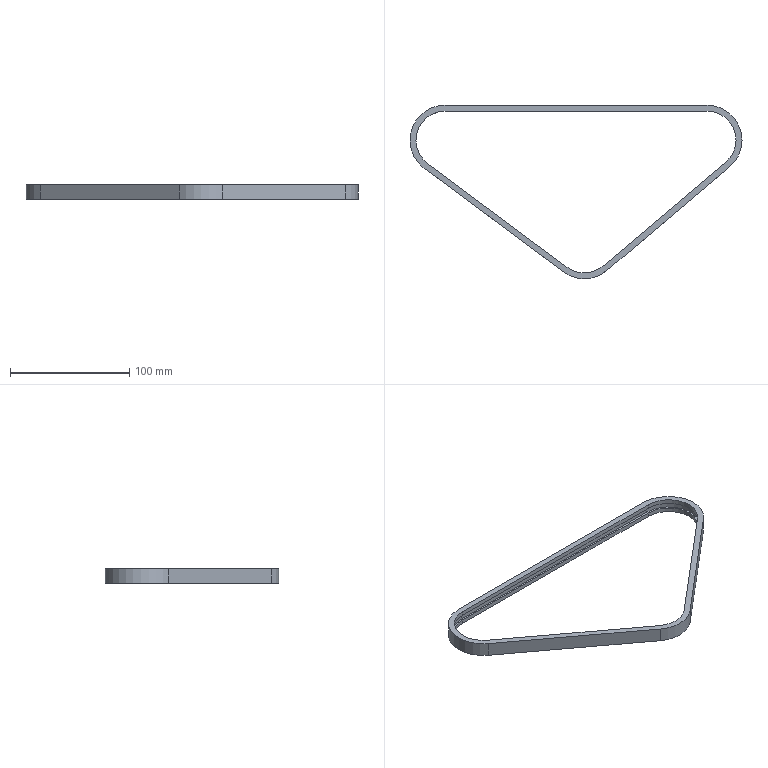Component | SolidWorks | LD101-02--Q1000-Q16-1.SLDQ1SM-1_LD101-02-Chain35B-1 | 1 solid | 32 faces | box 278.82 x 145.82 x 12 mm | volume 35184 mm3 | cylinder 16 | plane 16 | commonest cylinder face diameters 48.82 x8 52 x4 58.82 x4 | material 45
build123d program:
from build123d import *

# Parameters (mm, degrees)
EXTRUDE_THIN1_DEPTH            = 6
CHAIN_PLATE_GAP_SPROCKET_DEPTH = 2.385


with BuildPart() as part:
    # Sketch1_2 → Extrude-Thin1 (new, symmetric)
    with BuildSketch(Plane.XY):
        with BuildLine():
            Line((10.549, -110.6), (127.549, -23.6))
            ThreePointArc((127.549, -23.6), (137.92, 9.243), (110, 29.41))
            Line((110, 29.41), (-110, 29.41))
            ThreePointArc((-110, 29.41), (-137.62, 10.104), (-128.978, -22.468))
            Line((-128.978, -22.468), (-25.978, -109.468))
            ThreePointArc((-25.978, -109.468), (-7.912, -116.396), (10.549, -110.6))
        make_face()
        with BuildLine():
            Line((7.566, -106.588), (124.566, -19.588))
            ThreePointArc((124.566, -19.588), (133.173, 7.671), (110, 24.41))
            Line((110, 24.41), (-110, 24.41))
            ThreePointArc((-110, 24.41), (-132.924, 8.386), (-125.751, -18.648))
            Line((-125.751, -18.648), (-22.751, -105.648))
            ThreePointArc((-22.751, -105.648), (-7.757, -111.398), (7.566, -106.588))
        make_face(mode=Mode.SUBTRACT)
    extrude(amount=EXTRUDE_THIN1_DEPTH, both=True)

    # Sketch1_2 2 → Chain Plate Gap-Sprocket (cut, symmetric)
    with BuildSketch(Plane.XY):
        with BuildLine():
            Line((8.514, -107.864), (125.514, -20.864))
            ThreePointArc((125.514, -20.864), (134.683, 8.171), (110, 26))
            Line((110, 26), (-110, 26))
            ThreePointArc((-110, 26), (-134.418, 8.932), (-126.777, -19.863))
            Line((-126.777, -19.863), (-23.777, -106.863))
            ThreePointArc((-23.777, -106.863), (-7.806, -112.988), (8.514, -107.864))
        make_face()
        with BuildLine():
            Line((6.617, -105.312), (123.617, -18.312))
            ThreePointArc((123.617, -18.312), (131.664, 7.172), (110, 22.82))
            Line((110, 22.82), (-110, 22.82))
            ThreePointArc((-110, 22.82), (-131.431, 7.84), (-124.725, -17.433))
            Line((-124.725, -17.433), (-21.725, -104.433))
            ThreePointArc((-21.725, -104.433), (-7.707, -109.809), (6.617, -105.312))
        make_face(mode=Mode.SUBTRACT)
    extrude(amount=CHAIN_PLATE_GAP_SPROCKET_DEPTH, both=True, mode=Mode.SUBTRACT)


solid = part.part

# Placed as in the assembly
solid = solid.moved(Location((-760.29, 11.103, -50.893), (-180, 0, 180)))
STEP:
#1=COLOUR_RGB('',0.7922,0.8196,0.9333);
#2=FILL_AREA_STYLE_COLOUR('',#1);
#3=FILL_AREA_STYLE('',(#2));
#4=SURFACE_STYLE_FILL_AREA(#3);
#5=SURFACE_SIDE_STYLE('',(#4));
#6=SURFACE_STYLE_USAGE(.BOTH.,#5);
#7=PRESENTATION_STYLE_ASSIGNMENT((#6));
#8=CARTESIAN_POINT('',(-35.287,0.4371,-1.91));
#9=VERTEX_POINT('',#8);
#10=CARTESIAN_POINT('',(-34.263,1.461,-1.91));
#11=VERTEX_POINT('',#10);
#12=CARTESIAN_POINT('',(-34.263,0.4371,-1.91));
#13=DIRECTION('',(0.,0.,-1.));
#14=DIRECTION('',(-1.,-0.,-0.));
#15=AXIS2_PLACEMENT_3D('',#12,#13,#14);
#16=CIRCLE('',#15,1.024);
#17=EDGE_CURVE('',#9,#11,#16,.T.);
#18=ORIENTED_EDGE('',*,*,#17,.F.);
#19=CARTESIAN_POINT('',(-35.287,0.4371,-2.098));
#20=VERTEX_POINT('',#19);
#21=CARTESIAN_POINT('',(-35.287,0.4371,-1.91));
#22=DIRECTION('',(0.,0.,-1.));
#23=VECTOR('',#22,39.37);
#24=LINE('',#21,#23);
#25=EDGE_CURVE('',#9,#20,#24,.T.);
#26=ORIENTED_EDGE('',*,*,#25,.T.);
#27=CARTESIAN_POINT('',(-34.263,1.461,-2.098));
#28=VERTEX_POINT('',#27);
#29=CARTESIAN_POINT('',(-34.263,0.4371,-2.098));
#30=DIRECTION('',(0.,0.,-1.));
#31=DIRECTION('',(-1.,-0.,-0.));
#32=AXIS2_PLACEMENT_3D('',#29,#30,#31);
#33=CIRCLE('',#32,1.024);
#34=EDGE_CURVE('',#20,#28,#33,.T.);
#35=ORIENTED_EDGE('',*,*,#34,.T.);
#36=CARTESIAN_POINT('',(-34.263,1.461,-1.91));
#37=DIRECTION('',(0.,0.,-1.));
#38=VECTOR('',#37,39.37);
#39=LINE('',#36,#38);
#40=EDGE_CURVE('',#11,#28,#39,.T.);
#41=ORIENTED_EDGE('',*,*,#40,.F.);
#42=EDGE_LOOP('',(#18,#26,#35,#41));
#43=FACE_OUTER_BOUND('',#42,.T.);
#44=CARTESIAN_POINT('',(-34.263,0.4371,-1.91));
#45=DIRECTION('',(0.,0.,-1.));
#46=DIRECTION('',(-1.,-0.,-0.));
#47=AXIS2_PLACEMENT_3D('',#44,#45,#46);
#48=CYLINDRICAL_SURFACE('',#47,1.024);
#49=ADVANCED_FACE('',(#43),#48,.F.);
#50=CARTESIAN_POINT('',(-25.602,1.398,-2.24));
#51=VERTEX_POINT('',#50);
#52=CARTESIAN_POINT('',(-24.641,0.4371,-2.24));
#53=VERTEX_POINT('',#52);
#54=CARTESIAN_POINT('',(-25.602,0.4371,-2.24));
#55=DIRECTION('',(0.,0.,-1.));
#56=DIRECTION('',(-1.,-0.,-0.));
#57=AXIS2_PLACEMENT_3D('',#54,#55,#56);
#58=CIRCLE('',#57,0.961);
#59=EDGE_CURVE('',#51,#53,#58,.T.);
#60=ORIENTED_EDGE('',*,*,#59,.T.);
#61=CARTESIAN_POINT('',(-24.641,0.4371,-2.098));
#62=VERTEX_POINT('',#61);
#63=CARTESIAN_POINT('',(-24.641,0.4371,-2.24));
#64=DIRECTION('',(-0.,-0.,1.));
#65=VECTOR('',#64,39.37);
#66=LINE('',#63,#65);
#67=EDGE_CURVE('',#53,#62,#66,.T.);
#68=ORIENTED_EDGE('',*,*,#67,.T.);
#69=CARTESIAN_POINT('',(-25.602,1.398,-2.098));
#70=VERTEX_POINT('',#69);
#71=CARTESIAN_POINT('',(-25.602,0.4371,-2.098));
#72=DIRECTION('',(0.,0.,-1.));
#73=DIRECTION('',(-1.,-0.,-0.));
#74=AXIS2_PLACEMENT_3D('',#71,#72,#73);
#75=CIRCLE('',#74,0.961);
#76=EDGE_CURVE('',#70,#62,#75,.T.);
#77=ORIENTED_EDGE('',*,*,#76,.F.);
#78=CARTESIAN_POINT('',(-25.602,1.398,-2.24));
#79=DIRECTION('',(-0.,-0.,1.));
#80=VECTOR('',#79,39.37);
#81=LINE('',#78,#80);
#82=EDGE_CURVE('',#51,#70,#81,.T.);
#83=ORIENTED_EDGE('',*,*,#82,.F.);
#84=EDGE_LOOP('',(#60,#68,#77,#83));
#85=FACE_OUTER_BOUND('',#84,.T.);
#86=CARTESIAN_POINT('',(-25.602,0.4371,-2.24));
#87=DIRECTION('',(-0.,-0.,1.));
#88=DIRECTION('',(1.,0.,0.));
#89=AXIS2_PLACEMENT_3D('',#86,#87,#88);
#90=CYLINDRICAL_SURFACE('',#89,0.961);
#91=ADVANCED_FACE('',(#85),#90,.F.);
#92=CARTESIAN_POINT('',(-24.444,0.4371,-2.24));
#93=VERTEX_POINT('',#92);
#94=CARTESIAN_POINT('',(-24.855,-0.4474,-2.24));
#95=VERTEX_POINT('',#94);
#96=CARTESIAN_POINT('',(-25.602,0.4371,-2.24));
#97=DIRECTION('',(0.,0.,-1.));
#98=DIRECTION('',(-1.,-0.,-0.));
#99=AXIS2_PLACEMENT_3D('',#96,#97,#98);
#100=CIRCLE('',#99,1.158);
#101=EDGE_CURVE('',#93,#95,#100,.T.);
#102=ORIENTED_EDGE('',*,*,#101,.F.);
#103=CARTESIAN_POINT('',(-24.444,0.4371,-1.767));
#104=VERTEX_POINT('',#103);
#105=CARTESIAN_POINT('',(-24.444,0.4371,-2.24));
#106=DIRECTION('',(-0.,-0.,1.));
#107=VECTOR('',#106,39.37);
#108=LINE('',#105,#107);
#109=EDGE_CURVE('',#93,#104,#108,.T.);
#110=ORIENTED_EDGE('',*,*,#109,.T.);
#111=CARTESIAN_POINT('',(-24.855,-0.4474,-1.767));
#112=VERTEX_POINT('',#111);
#113=CARTESIAN_POINT('',(-25.602,0.4371,-1.767));
#114=DIRECTION('',(0.,0.,-1.));
#115=DIRECTION('',(-1.,-0.,-0.));
#116=AXIS2_PLACEMENT_3D('',#113,#114,#115);
#117=CIRCLE('',#116,1.158);
#118=EDGE_CURVE('',#104,#112,#117,.T.);
#119=ORIENTED_EDGE('',*,*,#118,.T.);
#120=CARTESIAN_POINT('',(-24.855,-0.4474,-2.24));
#121=DIRECTION('',(-0.,-0.,1.));
#122=VECTOR('',#121,39.37);
#123=LINE('',#120,#122);
#124=EDGE_CURVE('',#95,#112,#123,.T.);
#125=ORIENTED_EDGE('',*,*,#124,.F.);
#126=EDGE_LOOP('',(#102,#110,#119,#125));
#127=FACE_OUTER_BOUND('',#126,.T.);
#128=CARTESIAN_POINT('',(-25.602,0.4371,-2.24));
#129=DIRECTION('',(-0.,-0.,1.));
#130=DIRECTION('',(1.,0.,0.));
#131=AXIS2_PLACEMENT_3D('',#128,#129,#130);
#132=CYLINDRICAL_SURFACE('',#131,1.158);
#133=ADVANCED_FACE('',(#127),#132,.T.);
#134=CARTESIAN_POINT('',(-25.602,1.398,-1.91));
#135=VERTEX_POINT('',#134);
#136=CARTESIAN_POINT('',(-24.641,0.4371,-1.91));
#137=VERTEX_POINT('',#136);
#138=CARTESIAN_POINT('',(-25.602,0.4371,-1.91));
#139=DIRECTION('',(0.,0.,-1.));
#140=DIRECTION('',(-1.,-0.,-0.));
#141=AXIS2_PLACEMENT_3D('',#138,#139,#140);
#142=CIRCLE('',#141,0.961);
#143=EDGE_CURVE('',#135,#137,#142,.T.);
#144=ORIENTED_EDGE('',*,*,#143,.T.);
#145=CARTESIAN_POINT('',(-24.641,0.4371,-1.767));
#146=VERTEX_POINT('',#145);
#147=CARTESIAN_POINT('',(-24.641,0.4371,-2.24));
#148=DIRECTION('',(-0.,-0.,1.));
#149=VECTOR('',#148,39.37);
#150=LINE('',#147,#149);
#151=EDGE_CURVE('',#137,#146,#150,.T.);
#152=ORIENTED_EDGE('',*,*,#151,.T.);
#153=CARTESIAN_POINT('',(-25.602,1.398,-1.767));
#154=VERTEX_POINT('',#153);
#155=CARTESIAN_POINT('',(-25.602,0.4371,-1.767));
#156=DIRECTION('',(0.,0.,-1.));
#157=DIRECTION('',(-1.,-0.,-0.));
#158=AXIS2_PLACEMENT_3D('',#155,#156,#157);
#159=CIRCLE('',#158,0.961);
#160=EDGE_CURVE('',#154,#146,#159,.T.);
#161=ORIENTED_EDGE('',*,*,#160,.F.);
#162=CARTESIAN_POINT('',(-25.602,1.398,-2.24));
#163=DIRECTION('',(-0.,-0.,1.));
#164=VECTOR('',#163,39.37);
#165=LINE('',#162,#164);
#166=EDGE_CURVE('',#135,#154,#165,.T.);
#167=ORIENTED_EDGE('',*,*,#166,.F.);
#168=EDGE_LOOP('',(#144,#152,#161,#167));
#169=FACE_OUTER_BOUND('',#168,.T.);
#170=CARTESIAN_POINT('',(-25.602,0.4371,-2.24));
#171=DIRECTION('',(-0.,-0.,1.));
#172=DIRECTION('',(1.,0.,0.));
#173=AXIS2_PLACEMENT_3D('',#170,#171,#172);
#174=CYLINDRICAL_SURFACE('',#173,0.961);
#175=ADVANCED_FACE('',(#169),#174,.F.);
#176=CARTESIAN_POINT('',(-29.037,-3.722,-1.91));
#177=VERTEX_POINT('',#176);
#178=CARTESIAN_POINT('',(-29.037,-3.722,-1.767));
#179=VERTEX_POINT('',#178);
#180=CARTESIAN_POINT('',(-29.037,-3.722,-2.24));
#181=DIRECTION('',(-0.,-0.,1.));
#182=VECTOR('',#181,39.37);
#183=LINE('',#180,#182);
#184=EDGE_CURVE('',#177,#179,#183,.T.);
#185=ORIENTED_EDGE('',*,*,#184,.F.);
#186=CARTESIAN_POINT('',(-30.231,-3.759,-1.91));
#187=VERTEX_POINT('',#186);
#188=CARTESIAN_POINT('',(-29.657,-2.988,-1.91));
#189=DIRECTION('',(0.,0.,-1.));
#190=DIRECTION('',(-1.,0.,-0.));
#191=AXIS2_PLACEMENT_3D('',#188,#189,#190);
#192=CIRCLE('',#191,0.961);
#193=EDGE_CURVE('',#177,#187,#192,.T.);
#194=ORIENTED_EDGE('',*,*,#193,.T.);
#195=CARTESIAN_POINT('',(-30.231,-3.759,-1.767));
#196=VERTEX_POINT('',#195);
#197=CARTESIAN_POINT('',(-30.231,-3.759,-2.24));
#198=DIRECTION('',(-0.,-0.,1.));
#199=VECTOR('',#198,39.37);
#200=LINE('',#197,#199);
#201=EDGE_CURVE('',#187,#196,#200,.T.);
#202=ORIENTED_EDGE('',*,*,#201,.T.);
#203=CARTESIAN_POINT('',(-29.657,-2.988,-1.767));
#204=DIRECTION('',(0.,0.,-1.));
#205=DIRECTION('',(-1.,0.,-0.));
#206=AXIS2_PLACEMENT_3D('',#203,#204,#205);
#207=CIRCLE('',#206,0.961);
#208=EDGE_CURVE('',#179,#196,#207,.T.);
#209=ORIENTED_EDGE('',*,*,#208,.F.);
#210=EDGE_LOOP('',(#185,#194,#202,#209));
#211=FACE_OUTER_BOUND('',#210,.T.);
#212=CARTESIAN_POINT('',(-29.657,-2.988,-2.24));
#213=DIRECTION('',(-0.,-0.,1.));
#214=DIRECTION('',(1.,0.,0.));
#215=AXIS2_PLACEMENT_3D('',#212,#213,#214);
#216=CYLINDRICAL_SURFACE('',#215,0.961);
#217=ADVANCED_FACE('',(#211),#216,.F.);
#218=ORIENTED_EDGE('',*,*,#201,.F.);
#219=CARTESIAN_POINT('',(-34.837,-0.3341,-1.91));
#220=VERTEX_POINT('',#219);
#221=CARTESIAN_POINT('',(-30.231,-3.759,-1.91));
#222=DIRECTION('',(-0.8025,0.5967,-0.));
#223=VECTOR('',#222,39.37);
#224=LINE('',#221,#223);
#225=EDGE_CURVE('',#187,#220,#224,.T.);
#226=ORIENTED_EDGE('',*,*,#225,.T.);
#227=CARTESIAN_POINT('',(-34.837,-0.3341,-1.767));
#228=VERTEX_POINT('',#227);
#229=CARTESIAN_POINT('',(-34.837,-0.3341,-2.24));
#230=DIRECTION('',(-0.,-0.,1.));
#231=VECTOR('',#230,39.37);
#232=LINE('',#229,#231);
#233=EDGE_CURVE('',#220,#228,#232,.T.);
#234=ORIENTED_EDGE('',*,*,#233,.T.);
#235=CARTESIAN_POINT('',(-30.231,-3.759,-1.767));
#236=DIRECTION('',(-0.8025,0.5967,-0.));
#237=VECTOR('',#236,39.37);
#238=LINE('',#235,#237);
#239=EDGE_CURVE('',#196,#228,#238,.T.);
#240=ORIENTED_EDGE('',*,*,#239,.F.);
#241=EDGE_LOOP('',(#218,#226,#234,#240));
#242=FACE_OUTER_BOUND('',#241,.T.);
#243=CARTESIAN_POINT('',(-30.231,-3.759,-2.24));
#244=DIRECTION('',(0.5967,0.8025,0.));
#245=DIRECTION('',(0.8025,-0.5967,0.));
#246=AXIS2_PLACEMENT_3D('',#243,#244,#245);
#247=PLANE('',#246);
#248=ADVANCED_FACE('',(#242),#247,.T.);
#249=ORIENTED_EDGE('',*,*,#233,.F.);
#250=CARTESIAN_POINT('',(-34.263,1.398,-1.91));
#251=VERTEX_POINT('',#250);
#252=CARTESIAN_POINT('',(-34.263,0.4371,-1.91));
#253=DIRECTION('',(0.,0.,-1.));
#254=DIRECTION('',(-1.,-0.,-0.));
#255=AXIS2_PLACEMENT_3D('',#252,#253,#254);
#256=CIRCLE('',#255,0.961);
#257=EDGE_CURVE('',#220,#251,#256,.T.);
#258=ORIENTED_EDGE('',*,*,#257,.T.);
#259=CARTESIAN_POINT('',(-34.263,1.398,-1.767));
#260=VERTEX_POINT('',#259);
#261=CARTESIAN_POINT('',(-34.263,1.398,-2.24));
#262=DIRECTION('',(-0.,-0.,1.));
#263=VECTOR('',#262,39.37);
#264=LINE('',#261,#263);
#265=EDGE_CURVE('',#251,#260,#264,.T.);
#266=ORIENTED_EDGE('',*,*,#265,.T.);
#267=CARTESIAN_POINT('',(-34.263,0.4371,-1.767));
#268=DIRECTION('',(0.,0.,-1.));
#269=DIRECTION('',(1.,0.,0.));
#270=AXIS2_PLACEMENT_3D('',#267,#268,#269);
#271=CIRCLE('',#270,0.961);
#272=EDGE_CURVE('',#228,#260,#271,.T.);
#273=ORIENTED_EDGE('',*,*,#272,.F.);
#274=EDGE_LOOP('',(#249,#258,#266,#273));
#275=FACE_OUTER_BOUND('',#274,.T.);
#276=CARTESIAN_POINT('',(-34.263,0.4371,-2.24));
#277=DIRECTION('',(-0.,-0.,1.));
#278=DIRECTION('',(1.,0.,0.));
#279=AXIS2_PLACEMENT_3D('',#276,#277,#278);
#280=CYLINDRICAL_SURFACE('',#279,0.961);
#281=ADVANCED_FACE('',(#275),#280,.F.);
#282=ORIENTED_EDGE('',*,*,#265,.F.);
#283=CARTESIAN_POINT('',(-34.263,1.398,-1.91));
#284=DIRECTION('',(1.,0.,0.));
#285=VECTOR('',#284,39.37);
#286=LINE('',#283,#285);
#287=EDGE_CURVE('',#251,#135,#286,.T.);
#288=ORIENTED_EDGE('',*,*,#287,.T.);
#289=ORIENTED_EDGE('',*,*,#166,.T.);
#290=CARTESIAN_POINT('',(-34.263,1.398,-1.767));
#291=DIRECTION('',(1.,0.,0.));
#292=VECTOR('',#291,39.37);
#293=LINE('',#290,#292);
#294=EDGE_CURVE('',#260,#154,#293,.T.);
#295=ORIENTED_EDGE('',*,*,#294,.F.);
#296=EDGE_LOOP('',(#282,#288,#289,#295));
#297=FACE_OUTER_BOUND('',#296,.T.);
#298=CARTESIAN_POINT('',(-34.263,1.398,-2.24));
#299=DIRECTION('',(0.,-1.,-0.));
#300=DIRECTION('',(-0.,-0.,1.));
#301=AXIS2_PLACEMENT_3D('',#298,#299,#300);
#302=PLANE('',#301);
#303=ADVANCED_FACE('',(#297),#302,.T.);
#304=ORIENTED_EDGE('',*,*,#151,.F.);
#305=CARTESIAN_POINT('',(-24.982,-0.297,-1.91));
#306=VERTEX_POINT('',#305);
#307=CARTESIAN_POINT('',(-25.602,0.4371,-1.91));
#308=DIRECTION('',(0.,0.,-1.));
#309=DIRECTION('',(-1.,-0.,-0.));
#310=AXIS2_PLACEMENT_3D('',#307,#308,#309);
#311=CIRCLE('',#310,0.961);
#312=EDGE_CURVE('',#137,#306,#311,.T.);
#313=ORIENTED_EDGE('',*,*,#312,.T.);
#314=CARTESIAN_POINT('',(-24.982,-0.297,-1.767));
#315=VERTEX_POINT('',#314);
#316=CARTESIAN_POINT('',(-24.982,-0.297,-2.24));
#317=DIRECTION('',(-0.,-0.,1.));
#318=VECTOR('',#317,39.37);
#319=LINE('',#316,#318);
#320=EDGE_CURVE('',#306,#315,#319,.T.);
#321=ORIENTED_EDGE('',*,*,#320,.T.);
#322=CARTESIAN_POINT('',(-25.602,0.4371,-1.767));
#323=DIRECTION('',(0.,0.,-1.));
#324=DIRECTION('',(-1.,-0.,-0.));
#325=AXIS2_PLACEMENT_3D('',#322,#323,#324);
#326=CIRCLE('',#325,0.961);
#327=EDGE_CURVE('',#146,#315,#326,.T.);
#328=ORIENTED_EDGE('',*,*,#327,.F.);
#329=EDGE_LOOP('',(#304,#313,#321,#328));
#330=FACE_OUTER_BOUND('',#329,.T.);
#331=CARTESIAN_POINT('',(-25.602,0.4371,-2.24));
#332=DIRECTION('',(-0.,-0.,1.));
#333=DIRECTION('',(1.,0.,0.));
#334=AXIS2_PLACEMENT_3D('',#331,#332,#333);
#335=CYLINDRICAL_SURFACE('',#334,0.961);
#336=ADVANCED_FACE('',(#330),#335,.F.);
#337=ORIENTED_EDGE('',*,*,#320,.F.);
#338=CARTESIAN_POINT('',(-24.982,-0.297,-1.91));
#339=DIRECTION('',(-0.7639,-0.6453,-0.));
#340=VECTOR('',#339,39.37);
#341=LINE('',#338,#340);
#342=EDGE_CURVE('',#306,#177,#341,.T.);
#343=ORIENTED_EDGE('',*,*,#342,.T.);
#344=ORIENTED_EDGE('',*,*,#184,.T.);
#345=CARTESIAN_POINT('',(-24.982,-0.297,-1.767));
#346=DIRECTION('',(-0.7639,-0.6453,-0.));
#347=VECTOR('',#346,39.37);
#348=LINE('',#345,#347);
#349=EDGE_CURVE('',#315,#179,#348,.T.);
#350=ORIENTED_EDGE('',*,*,#349,.F.);
#351=EDGE_LOOP('',(#337,#343,#344,#350));
#352=FACE_OUTER_BOUND('',#351,.T.);
#353=CARTESIAN_POINT('',(-24.982,-0.297,-2.24));
#354=DIRECTION('',(-0.6453,0.7639,-0.));
#355=DIRECTION('',(0.7639,0.6453,0.));
#356=AXIS2_PLACEMENT_3D('',#353,#354,#355);
#357=PLANE('',#356);
#358=ADVANCED_FACE('',(#352),#357,.T.);
#359=CARTESIAN_POINT('',(-28.91,-3.873,-2.24));
#360=VERTEX_POINT('',#359);
#361=CARTESIAN_POINT('',(-30.348,-3.917,-2.24));
#362=VERTEX_POINT('',#361);
#363=CARTESIAN_POINT('',(-29.657,-2.988,-2.24));
#364=DIRECTION('',(0.,0.,-1.));
#365=DIRECTION('',(-1.,0.,-0.));
#366=AXIS2_PLACEMENT_3D('',#363,#364,#365);
#367=CIRCLE('',#366,1.158);
#368=EDGE_CURVE('',#360,#362,#367,.T.);
#369=ORIENTED_EDGE('',*,*,#368,.T.);
#370=CARTESIAN_POINT('',(-34.954,-0.492,-2.24));
#371=VERTEX_POINT('',#370);
#372=CARTESIAN_POINT('',(-30.348,-3.917,-2.24));
#373=DIRECTION('',(-0.8025,0.5967,-0.));
#374=VECTOR('',#373,39.37);
#375=LINE('',#372,#374);
#376=EDGE_CURVE('',#362,#371,#375,.T.);
#377=ORIENTED_EDGE('',*,*,#376,.T.);
#378=CARTESIAN_POINT('',(-34.263,1.595,-2.24));
#379=VERTEX_POINT('',#378);
#380=CARTESIAN_POINT('',(-34.263,0.4371,-2.24));
#381=DIRECTION('',(0.,0.,-1.));
#382=DIRECTION('',(-1.,-0.,-0.));
#383=AXIS2_PLACEMENT_3D('',#380,#381,#382);
#384=CIRCLE('',#383,1.158);
#385=EDGE_CURVE('',#371,#379,#384,.T.);
#386=ORIENTED_EDGE('',*,*,#385,.T.);
#387=CARTESIAN_POINT('',(-25.602,1.595,-2.24));
#388=VERTEX_POINT('',#387);
#389=CARTESIAN_POINT('',(-34.263,1.595,-2.24));
#390=DIRECTION('',(1.,0.,0.));
#391=VECTOR('',#390,39.37);
#392=LINE('',#389,#391);
#393=EDGE_CURVE('',#379,#388,#392,.T.);
#394=ORIENTED_EDGE('',*,*,#393,.T.);
#395=CARTESIAN_POINT('',(-25.602,0.4371,-2.24));
#396=DIRECTION('',(0.,0.,-1.));
#397=DIRECTION('',(-1.,-0.,-0.));
#398=AXIS2_PLACEMENT_3D('',#395,#396,#397);
#399=CIRCLE('',#398,1.158);
#400=EDGE_CURVE('',#388,#93,#399,.T.);
#401=ORIENTED_EDGE('',*,*,#400,.T.);
#402=ORIENTED_EDGE('',*,*,#101,.T.);
#403=CARTESIAN_POINT('',(-24.855,-0.4474,-2.24));
#404=DIRECTION('',(-0.7639,-0.6453,-0.));
#405=VECTOR('',#404,39.37);
#406=LINE('',#403,#405);
#407=EDGE_CURVE('',#95,#360,#406,.T.);
#408=ORIENTED_EDGE('',*,*,#407,.T.);
#409=EDGE_LOOP('',(#369,#377,#386,#394,#401,#402,#408));
#410=FACE_OUTER_BOUND('',#409,.T.);
#411=CARTESIAN_POINT('',(-30.231,-3.759,-2.24));
#412=VERTEX_POINT('',#411);
#413=CARTESIAN_POINT('',(-34.837,-0.3341,-2.24));
#414=VERTEX_POINT('',#413);
#415=CARTESIAN_POINT('',(-30.231,-3.759,-2.24));
#416=DIRECTION('',(-0.8025,0.5967,-0.));
#417=VECTOR('',#416,39.37);
#418=LINE('',#415,#417);
#419=EDGE_CURVE('',#412,#414,#418,.T.);
#420=ORIENTED_EDGE('',*,*,#419,.F.);
#421=CARTESIAN_POINT('',(-29.037,-3.722,-2.24));
#422=VERTEX_POINT('',#421);
#423=CARTESIAN_POINT('',(-29.657,-2.988,-2.24));
#424=DIRECTION('',(0.,0.,-1.));
#425=DIRECTION('',(-1.,0.,-0.));
#426=AXIS2_PLACEMENT_3D('',#423,#424,#425);
#427=CIRCLE('',#426,0.961);
#428=EDGE_CURVE('',#422,#412,#427,.T.);
#429=ORIENTED_EDGE('',*,*,#428,.F.);
#430=CARTESIAN_POINT('',(-24.982,-0.297,-2.24));
#431=VERTEX_POINT('',#430);
#432=CARTESIAN_POINT('',(-24.982,-0.297,-2.24));
#433=DIRECTION('',(-0.7639,-0.6453,-0.));
#434=VECTOR('',#433,39.37);
#435=LINE('',#432,#434);
#436=EDGE_CURVE('',#431,#422,#435,.T.);
#437=ORIENTED_EDGE('',*,*,#436,.F.);
#438=CARTESIAN_POINT('',(-25.602,0.4371,-2.24));
#439=DIRECTION('',(0.,0.,-1.));
#440=DIRECTION('',(-1.,-0.,-0.));
#441=AXIS2_PLACEMENT_3D('',#438,#439,#440);
#442=CIRCLE('',#441,0.961);
#443=EDGE_CURVE('',#53,#431,#442,.T.);
#444=ORIENTED_EDGE('',*,*,#443,.F.);
#445=ORIENTED_EDGE('',*,*,#59,.F.);
#446=CARTESIAN_POINT('',(-34.263,1.398,-2.24));
#447=VERTEX_POINT('',#446);
#448=CARTESIAN_POINT('',(-34.263,1.398,-2.24));
#449=DIRECTION('',(1.,0.,0.));
#450=VECTOR('',#449,39.37);
#451=LINE('',#448,#450);
#452=EDGE_CURVE('',#447,#51,#451,.T.);
#453=ORIENTED_EDGE('',*,*,#452,.F.);
#454=CARTESIAN_POINT('',(-34.263,0.4371,-2.24));
#455=DIRECTION('',(0.,0.,-1.));
#456=DIRECTION('',(1.,0.,0.));
#457=AXIS2_PLACEMENT_3D('',#454,#455,#456);
#458=CIRCLE('',#457,0.961);
#459=EDGE_CURVE('',#414,#447,#458,.T.);
#460=ORIENTED_EDGE('',*,*,#459,.F.);
#461=EDGE_LOOP('',(#420,#429,#437,#444,#445,#453,#460));
#462=FACE_BOUND('',#461,.T.);
#463=CARTESIAN_POINT('',(-29.657,-2.988,-2.24));
#464=DIRECTION('',(0.,0.,-1.));
#465=DIRECTION('',(-1.,-0.,-0.));
#466=AXIS2_PLACEMENT_3D('',#463,#464,#465);
#467=PLANE('',#466);
#468=ADVANCED_FACE('',(#410,#462),#467,.T.);
#469=CARTESIAN_POINT('',(-28.91,-3.873,-1.767));
#470=VERTEX_POINT('',#469);
#471=CARTESIAN_POINT('',(-30.348,-3.917,-1.767));
#472=VERTEX_POINT('',#471);
#473=CARTESIAN_POINT('',(-29.657,-2.988,-1.767));
#474=DIRECTION('',(0.,0.,-1.));
#475=DIRECTION('',(-1.,0.,-0.));
#476=AXIS2_PLACEMENT_3D('',#473,#474,#475);
#477=CIRCLE('',#476,1.158);
#478=EDGE_CURVE('',#470,#472,#477,.T.);
#479=ORIENTED_EDGE('',*,*,#478,.F.);
#480=CARTESIAN_POINT('',(-24.855,-0.4474,-1.767));
#481=DIRECTION('',(-0.7639,-0.6453,-0.));
#482=VECTOR('',#481,39.37);
#483=LINE('',#480,#482);
#484=EDGE_CURVE('',#112,#470,#483,.T.);
#485=ORIENTED_EDGE('',*,*,#484,.F.);
#486=ORIENTED_EDGE('',*,*,#118,.F.);
#487=CARTESIAN_POINT('',(-25.602,1.595,-1.767));
#488=VERTEX_POINT('',#487);
#489=CARTESIAN_POINT('',(-25.602,0.4371,-1.767));
#490=DIRECTION('',(0.,0.,-1.));
#491=DIRECTION('',(-1.,-0.,-0.));
#492=AXIS2_PLACEMENT_3D('',#489,#490,#491);
#493=CIRCLE('',#492,1.158);
#494=EDGE_CURVE('',#488,#104,#493,.T.);
#495=ORIENTED_EDGE('',*,*,#494,.F.);
#496=CARTESIAN_POINT('',(-34.263,1.595,-1.767));
#497=VERTEX_POINT('',#496);
#498=CARTESIAN_POINT('',(-34.263,1.595,-1.767));
#499=DIRECTION('',(1.,0.,0.));
#500=VECTOR('',#499,39.37);
#501=LINE('',#498,#500);
#502=EDGE_CURVE('',#497,#488,#501,.T.);
#503=ORIENTED_EDGE('',*,*,#502,.F.);
#504=CARTESIAN_POINT('',(-34.954,-0.492,-1.767));
#505=VERTEX_POINT('',#504);
#506=CARTESIAN_POINT('',(-34.263,0.4371,-1.767));
#507=DIRECTION('',(0.,0.,-1.));
#508=DIRECTION('',(-1.,-0.,-0.));
#509=AXIS2_PLACEMENT_3D('',#506,#507,#508);
#510=CIRCLE('',#509,1.158);
#511=EDGE_CURVE('',#505,#497,#510,.T.);
#512=ORIENTED_EDGE('',*,*,#511,.F.);
#513=CARTESIAN_POINT('',(-30.348,-3.917,-1.767));
#514=DIRECTION('',(-0.8025,0.5967,-0.));
#515=VECTOR('',#514,39.37);
#516=LINE('',#513,#515);
#517=EDGE_CURVE('',#472,#505,#516,.T.);
#518=ORIENTED_EDGE('',*,*,#517,.F.);
#519=EDGE_LOOP('',(#479,#485,#486,#495,#503,#512,#518));
#520=FACE_OUTER_BOUND('',#519,.T.);
#521=ORIENTED_EDGE('',*,*,#208,.T.);
#522=ORIENTED_EDGE('',*,*,#239,.T.);
#523=ORIENTED_EDGE('',*,*,#272,.T.);
#524=ORIENTED_EDGE('',*,*,#294,.T.);
#525=ORIENTED_EDGE('',*,*,#160,.T.);
#526=ORIENTED_EDGE('',*,*,#327,.T.);
#527=ORIENTED_EDGE('',*,*,#349,.T.);
#528=EDGE_LOOP('',(#521,#522,#523,#524,#525,#526,#527));
#529=FACE_BOUND('',#528,.T.);
#530=CARTESIAN_POINT('',(-29.657,-2.988,-1.767));
#531=DIRECTION('',(0.,0.,-1.));
#532=DIRECTION('',(-1.,-0.,-0.));
#533=AXIS2_PLACEMENT_3D('',#530,#531,#532);
#534=PLANE('',#533);
#535=ADVANCED_FACE('',(#520,#529),#534,.F.);
#536=ORIENTED_EDGE('',*,*,#478,.T.);
#537=CARTESIAN_POINT('',(-30.348,-3.917,-2.24));
#538=DIRECTION('',(-0.,-0.,1.));
#539=VECTOR('',#538,39.37);
#540=LINE('',#537,#539);
#541=EDGE_CURVE('',#362,#472,#540,.T.);
#542=ORIENTED_EDGE('',*,*,#541,.F.);
#543=ORIENTED_EDGE('',*,*,#368,.F.);
#544=CARTESIAN_POINT('',(-28.91,-3.873,-2.24));
#545=DIRECTION('',(-0.,-0.,1.));
#546=VECTOR('',#545,39.37);
#547=LINE('',#544,#546);
#548=EDGE_CURVE('',#360,#470,#547,.T.);
#549=ORIENTED_EDGE('',*,*,#548,.T.);
#550=EDGE_LOOP('',(#536,#542,#543,#549));
#551=FACE_OUTER_BOUND('',#550,.T.);
#552=CARTESIAN_POINT('',(-29.657,-2.988,-2.24));
#553=DIRECTION('',(-0.,-0.,1.));
#554=DIRECTION('',(1.,0.,0.));
#555=AXIS2_PLACEMENT_3D('',#552,#553,#554);
#556=CYLINDRICAL_SURFACE('',#555,1.158);
#557=ADVANCED_FACE('',(#551),#556,.T.);
#558=ORIENTED_EDGE('',*,*,#517,.T.);
#559=CARTESIAN_POINT('',(-34.954,-0.492,-2.24));
#560=DIRECTION('',(-0.,-0.,1.));
#561=VECTOR('',#560,39.37);
#562=LINE('',#559,#561);
#563=EDGE_CURVE('',#371,#505,#562,.T.);
#564=ORIENTED_EDGE('',*,*,#563,.F.);
#565=ORIENTED_EDGE('',*,*,#376,.F.);
#566=ORIENTED_EDGE('',*,*,#541,.T.);
#567=EDGE_LOOP('',(#558,#564,#565,#566));
#568=FACE_OUTER_BOUND('',#567,.T.);
#569=CARTESIAN_POINT('',(-30.348,-3.917,-2.24));
#570=DIRECTION('',(0.5967,0.8025,0.));
#571=DIRECTION('',(0.8025,-0.5967,0.));
#572=AXIS2_PLACEMENT_3D('',#569,#570,#571);
#573=PLANE('',#572);
#574=ADVANCED_FACE('',(#568),#573,.F.);
#575=ORIENTED_EDGE('',*,*,#511,.T.);
#576=CARTESIAN_POINT('',(-34.263,1.595,-2.24));
#577=DIRECTION('',(-0.,-0.,1.));
#578=VECTOR('',#577,39.37);
#579=LINE('',#576,#578);
#580=EDGE_CURVE('',#379,#497,#579,.T.);
#581=ORIENTED_EDGE('',*,*,#580,.F.);
#582=ORIENTED_EDGE('',*,*,#385,.F.);
#583=ORIENTED_EDGE('',*,*,#563,.T.);
#584=EDGE_LOOP('',(#575,#581,#582,#583));
#585=FACE_OUTER_BOUND('',#584,.T.);
#586=CARTESIAN_POINT('',(-34.263,0.4371,-2.24));
#587=DIRECTION('',(-0.,-0.,1.));
#588=DIRECTION('',(1.,0.,0.));
#589=AXIS2_PLACEMENT_3D('',#586,#587,#588);
#590=CYLINDRICAL_SURFACE('',#589,1.158);
#591=ADVANCED_FACE('',(#585),#590,.T.);
#592=ORIENTED_EDGE('',*,*,#502,.T.);
#593=CARTESIAN_POINT('',(-25.602,1.595,-2.24));
#594=DIRECTION('',(-0.,-0.,1.));
#595=VECTOR('',#594,39.37);
#596=LINE('',#593,#595);
#597=EDGE_CURVE('',#388,#488,#596,.T.);
#598=ORIENTED_EDGE('',*,*,#597,.F.);
#599=ORIENTED_EDGE('',*,*,#393,.F.);
#600=ORIENTED_EDGE('',*,*,#580,.T.);
#601=EDGE_LOOP('',(#592,#598,#599,#600));
#602=FACE_OUTER_BOUND('',#601,.T.);
#603=CARTESIAN_POINT('',(-34.263,1.595,-2.24));
#604=DIRECTION('',(0.,-1.,-0.));
#605=DIRECTION('',(-0.,-0.,1.));
#606=AXIS2_PLACEMENT_3D('',#603,#604,#605);
#607=PLANE('',#606);
#608=ADVANCED_FACE('',(#602),#607,.F.);
#609=ORIENTED_EDGE('',*,*,#109,.F.);
#610=ORIENTED_EDGE('',*,*,#400,.F.);
#611=ORIENTED_EDGE('',*,*,#597,.T.);
#612=ORIENTED_EDGE('',*,*,#494,.T.);
#613=EDGE_LOOP('',(#609,#610,#611,#612));
#614=FACE_OUTER_BOUND('',#613,.T.);
#615=CARTESIAN_POINT('',(-25.602,0.4371,-2.24));
#616=DIRECTION('',(-0.,-0.,1.));
#617=DIRECTION('',(1.,0.,0.));
#618=AXIS2_PLACEMENT_3D('',#615,#616,#617);
#619=CYLINDRICAL_SURFACE('',#618,1.158);
#620=ADVANCED_FACE('',(#614),#619,.T.);
#621=ORIENTED_EDGE('',*,*,#484,.T.);
#622=ORIENTED_EDGE('',*,*,#548,.F.);
#623=ORIENTED_EDGE('',*,*,#407,.F.);
#624=ORIENTED_EDGE('',*,*,#124,.T.);
#625=EDGE_LOOP('',(#621,#622,#623,#624));
#626=FACE_OUTER_BOUND('',#625,.T.);
#627=CARTESIAN_POINT('',(-24.855,-0.4474,-2.24));
#628=DIRECTION('',(-0.6453,0.7639,-0.));
#629=DIRECTION('',(0.7639,0.6453,0.));
#630=AXIS2_PLACEMENT_3D('',#627,#628,#629);
#631=PLANE('',#630);
#632=ADVANCED_FACE('',(#626),#631,.F.);
#633=CARTESIAN_POINT('',(-29.037,-3.722,-2.098));
#634=VERTEX_POINT('',#633);
#635=CARTESIAN_POINT('',(-30.231,-3.759,-2.098));
#636=VERTEX_POINT('',#635);
#637=CARTESIAN_POINT('',(-29.657,-2.988,-2.098));
#638=DIRECTION('',(0.,0.,-1.));
#639=DIRECTION('',(-1.,0.,-0.));
#640=AXIS2_PLACEMENT_3D('',#637,#638,#639);
#641=CIRCLE('',#640,0.961);
#642=EDGE_CURVE('',#634,#636,#641,.T.);
#643=ORIENTED_EDGE('',*,*,#642,.F.);
#644=CARTESIAN_POINT('',(-29.037,-3.722,-2.24));
#645=DIRECTION('',(-0.,-0.,1.));
#646=VECTOR('',#645,39.37);
#647=LINE('',#644,#646);
#648=EDGE_CURVE('',#422,#634,#647,.T.);
#649=ORIENTED_EDGE('',*,*,#648,.F.);
#650=ORIENTED_EDGE('',*,*,#428,.T.);
#651=CARTESIAN_POINT('',(-30.231,-3.759,-2.24));
#652=DIRECTION('',(-0.,-0.,1.));
#653=VECTOR('',#652,39.37);
#654=LINE('',#651,#653);
#655=EDGE_CURVE('',#412,#636,#654,.T.);
#656=ORIENTED_EDGE('',*,*,#655,.T.);
#657=EDGE_LOOP('',(#643,#649,#650,#656));
#658=FACE_OUTER_BOUND('',#657,.T.);
#659=CARTESIAN_POINT('',(-29.657,-2.988,-2.24));
#660=DIRECTION('',(-0.,-0.,1.));
#661=DIRECTION('',(1.,0.,0.));
#662=AXIS2_PLACEMENT_3D('',#659,#660,#661);
#663=CYLINDRICAL_SURFACE('',#662,0.961);
#664=ADVANCED_FACE('',(#658),#663,.F.);
#665=CARTESIAN_POINT('',(-34.837,-0.3341,-2.098));
#666=VERTEX_POINT('',#665);
#667=CARTESIAN_POINT('',(-30.231,-3.759,-2.098));
#668=DIRECTION('',(-0.8025,0.5967,-0.));
#669=VECTOR('',#668,39.37);
#670=LINE('',#667,#669);
#671=EDGE_CURVE('',#636,#666,#670,.T.);
#672=ORIENTED_EDGE('',*,*,#671,.F.);
#673=ORIENTED_EDGE('',*,*,#655,.F.);
#674=ORIENTED_EDGE('',*,*,#419,.T.);
#675=CARTESIAN_POINT('',(-34.837,-0.3341,-2.24));
#676=DIRECTION('',(-0.,-0.,1.));
#677=VECTOR('',#676,39.37);
#678=LINE('',#675,#677);
#679=EDGE_CURVE('',#414,#666,#678,.T.);
#680=ORIENTED_EDGE('',*,*,#679,.T.);
#681=EDGE_LOOP('',(#672,#673,#674,#680));
#682=FACE_OUTER_BOUND('',#681,.T.);
#683=CARTESIAN_POINT('',(-30.231,-3.759,-2.24));
#684=DIRECTION('',(0.5967,0.8025,0.));
#685=DIRECTION('',(0.8025,-0.5967,0.));
#686=AXIS2_PLACEMENT_3D('',#683,#684,#685);
#687=PLANE('',#686);
#688=ADVANCED_FACE('',(#682),#687,.T.);
#689=CARTESIAN_POINT('',(-34.263,1.398,-2.098));
#690=VERTEX_POINT('',#689);
#691=CARTESIAN_POINT('',(-34.263,0.4371,-2.098));
#692=DIRECTION('',(0.,0.,-1.));
#693=DIRECTION('',(-1.,-0.,-0.));
#694=AXIS2_PLACEMENT_3D('',#691,#692,#693);
#695=CIRCLE('',#694,0.961);
#696=EDGE_CURVE('',#666,#690,#695,.T.);
#697=ORIENTED_EDGE('',*,*,#696,.F.);
#698=ORIENTED_EDGE('',*,*,#679,.F.);
#699=ORIENTED_EDGE('',*,*,#459,.T.);
#700=CARTESIAN_POINT('',(-34.263,1.398,-2.24));
#701=DIRECTION('',(-0.,-0.,1.));
#702=VECTOR('',#701,39.37);
#703=LINE('',#700,#702);
#704=EDGE_CURVE('',#447,#690,#703,.T.);
#705=ORIENTED_EDGE('',*,*,#704,.T.);
#706=EDGE_LOOP('',(#697,#698,#699,#705));
#707=FACE_OUTER_BOUND('',#706,.T.);
#708=CARTESIAN_POINT('',(-34.263,0.4371,-2.24));
#709=DIRECTION('',(-0.,-0.,1.));
#710=DIRECTION('',(1.,0.,0.));
#711=AXIS2_PLACEMENT_3D('',#708,#709,#710);
#712=CYLINDRICAL_SURFACE('',#711,0.961);
#713=ADVANCED_FACE('',(#707),#712,.F.);
#714=CARTESIAN_POINT('',(-34.263,1.398,-2.098));
#715=DIRECTION('',(1.,0.,0.));
#716=VECTOR('',#715,39.37);
#717=LINE('',#714,#716);
#718=EDGE_CURVE('',#690,#70,#717,.T.);
#719=ORIENTED_EDGE('',*,*,#718,.F.);
#720=ORIENTED_EDGE('',*,*,#704,.F.);
#721=ORIENTED_EDGE('',*,*,#452,.T.);
#722=ORIENTED_EDGE('',*,*,#82,.T.);
#723=EDGE_LOOP('',(#719,#720,#721,#722));
#724=FACE_OUTER_BOUND('',#723,.T.);
#725=CARTESIAN_POINT('',(-34.263,1.398,-2.24));
#726=DIRECTION('',(0.,-1.,-0.));
#727=DIRECTION('',(-0.,-0.,1.));
#728=AXIS2_PLACEMENT_3D('',#725,#726,#727);
#729=PLANE('',#728);
#730=ADVANCED_FACE('',(#724),#729,.T.);
#731=ORIENTED_EDGE('',*,*,#67,.F.);
#732=ORIENTED_EDGE('',*,*,#443,.T.);
#733=CARTESIAN_POINT('',(-24.982,-0.297,-2.098));
#734=VERTEX_POINT('',#733);
#735=CARTESIAN_POINT('',(-24.982,-0.297,-2.24));
#736=DIRECTION('',(-0.,-0.,1.));
#737=VECTOR('',#736,39.37);
#738=LINE('',#735,#737);
#739=EDGE_CURVE('',#431,#734,#738,.T.);
#740=ORIENTED_EDGE('',*,*,#739,.T.);
#741=CARTESIAN_POINT('',(-25.602,0.4371,-2.098));
#742=DIRECTION('',(0.,0.,-1.));
#743=DIRECTION('',(-1.,-0.,-0.));
#744=AXIS2_PLACEMENT_3D('',#741,#742,#743);
#745=CIRCLE('',#744,0.961);
#746=EDGE_CURVE('',#62,#734,#745,.T.);
#747=ORIENTED_EDGE('',*,*,#746,.F.);
#748=EDGE_LOOP('',(#731,#732,#740,#747));
#749=FACE_OUTER_BOUND('',#748,.T.);
#750=CARTESIAN_POINT('',(-25.602,0.4371,-2.24));
#751=DIRECTION('',(-0.,-0.,1.));
#752=DIRECTION('',(1.,0.,0.));
#753=AXIS2_PLACEMENT_3D('',#750,#751,#752);
#754=CYLINDRICAL_SURFACE('',#753,0.961);
#755=ADVANCED_FACE('',(#749),#754,.F.);
#756=CARTESIAN_POINT('',(-24.982,-0.297,-2.098));
#757=DIRECTION('',(-0.7639,-0.6453,-0.));
#758=VECTOR('',#757,39.37);
#759=LINE('',#756,#758);
#760=EDGE_CURVE('',#734,#634,#759,.T.);
#761=ORIENTED_EDGE('',*,*,#760,.F.);
#762=ORIENTED_EDGE('',*,*,#739,.F.);
#763=ORIENTED_EDGE('',*,*,#436,.T.);
#764=ORIENTED_EDGE('',*,*,#648,.T.);
#765=EDGE_LOOP('',(#761,#762,#763,#764));
#766=FACE_OUTER_BOUND('',#765,.T.);
#767=CARTESIAN_POINT('',(-24.982,-0.297,-2.24));
#768=DIRECTION('',(-0.6453,0.7639,-0.));
#769=DIRECTION('',(0.7639,0.6453,0.));
#770=AXIS2_PLACEMENT_3D('',#767,#768,#769);
#771=PLANE('',#770);
#772=ADVANCED_FACE('',(#766),#771,.T.);
#773=CARTESIAN_POINT('',(-28.997,-3.77,-2.098));
#774=VERTEX_POINT('',#773);
#775=CARTESIAN_POINT('',(-30.268,-3.809,-2.098));
#776=VERTEX_POINT('',#775);
#777=CARTESIAN_POINT('',(-29.657,-2.988,-2.098));
#778=DIRECTION('',(0.,0.,-1.));
#779=DIRECTION('',(-1.,0.,-0.));
#780=AXIS2_PLACEMENT_3D('',#777,#778,#779);
#781=CIRCLE('',#780,1.024);
#782=EDGE_CURVE('',#774,#776,#781,.T.);
#783=ORIENTED_EDGE('',*,*,#782,.T.);
#784=CARTESIAN_POINT('',(-30.268,-3.809,-1.91));
#785=VERTEX_POINT('',#784);
#786=CARTESIAN_POINT('',(-30.268,-3.809,-1.91));
#787=DIRECTION('',(0.,0.,-1.));
#788=VECTOR('',#787,39.37);
#789=LINE('',#786,#788);
#790=EDGE_CURVE('',#785,#776,#789,.T.);
#791=ORIENTED_EDGE('',*,*,#790,.F.);
#792=CARTESIAN_POINT('',(-28.997,-3.77,-1.91));
#793=VERTEX_POINT('',#792);
#794=CARTESIAN_POINT('',(-29.657,-2.988,-1.91));
#795=DIRECTION('',(0.,0.,-1.));
#796=DIRECTION('',(-1.,0.,-0.));
#797=AXIS2_PLACEMENT_3D('',#794,#795,#796);
#798=CIRCLE('',#797,1.024);
#799=EDGE_CURVE('',#793,#785,#798,.T.);
#800=ORIENTED_EDGE('',*,*,#799,.F.);
#801=CARTESIAN_POINT('',(-28.997,-3.77,-1.91));
#802=DIRECTION('',(0.,0.,-1.));
#803=VECTOR('',#802,39.37);
#804=LINE('',#801,#803);
#805=EDGE_CURVE('',#793,#774,#804,.T.);
#806=ORIENTED_EDGE('',*,*,#805,.T.);
#807=EDGE_LOOP('',(#783,#791,#800,#806));
#808=FACE_OUTER_BOUND('',#807,.T.);
#809=CARTESIAN_POINT('',(-29.657,-2.988,-1.91));
#810=DIRECTION('',(0.,0.,-1.));
#811=DIRECTION('',(-1.,0.,-0.));
#812=AXIS2_PLACEMENT_3D('',#809,#810,#811);
#813=CYLINDRICAL_SURFACE('',#812,1.024);
#814=ADVANCED_FACE('',(#808),#813,.F.);
#815=CARTESIAN_POINT('',(-24.941,-0.3449,-2.098));
#816=VERTEX_POINT('',#815);
#817=CARTESIAN_POINT('',(-24.941,-0.3449,-2.098));
#818=DIRECTION('',(-0.7639,-0.6453,-0.));
#819=VECTOR('',#818,39.37);
#820=LINE('',#817,#819);
#821=EDGE_CURVE('',#816,#774,#820,.T.);
#822=ORIENTED_EDGE('',*,*,#821,.T.);
#823=ORIENTED_EDGE('',*,*,#805,.F.);
#824=CARTESIAN_POINT('',(-24.941,-0.3449,-1.91));
#825=VERTEX_POINT('',#824);
#826=CARTESIAN_POINT('',(-24.941,-0.3449,-1.91));
#827=DIRECTION('',(-0.7639,-0.6453,-0.));
#828=VECTOR('',#827,39.37);
#829=LINE('',#826,#828);
#830=EDGE_CURVE('',#825,#793,#829,.T.);
#831=ORIENTED_EDGE('',*,*,#830,.F.);
#832=CARTESIAN_POINT('',(-24.941,-0.3449,-1.91));
#833=DIRECTION('',(0.,0.,-1.));
#834=VECTOR('',#833,39.37);
#835=LINE('',#832,#834);
#836=EDGE_CURVE('',#825,#816,#835,.T.);
#837=ORIENTED_EDGE('',*,*,#836,.T.);
#838=EDGE_LOOP('',(#822,#823,#831,#837));
#839=FACE_OUTER_BOUND('',#838,.T.);
#840=CARTESIAN_POINT('',(-24.941,-0.3449,-1.91));
#841=DIRECTION('',(0.6453,-0.7639,0.));
#842=DIRECTION('',(-0.7639,-0.6453,-0.));
#843=AXIS2_PLACEMENT_3D('',#840,#841,#842);
#844=PLANE('',#843);
#845=ADVANCED_FACE('',(#839),#844,.F.);
#846=CARTESIAN_POINT('',(-25.602,1.461,-2.098));
#847=VERTEX_POINT('',#846);
#848=CARTESIAN_POINT('',(-25.602,0.4371,-2.098));
#849=DIRECTION('',(0.,0.,-1.));
#850=DIRECTION('',(-1.,-0.,-0.));
#851=AXIS2_PLACEMENT_3D('',#848,#849,#850);
#852=CIRCLE('',#851,1.024);
#853=EDGE_CURVE('',#847,#816,#852,.T.);
#854=ORIENTED_EDGE('',*,*,#853,.T.);
#855=ORIENTED_EDGE('',*,*,#836,.F.);
#856=CARTESIAN_POINT('',(-25.602,1.461,-1.91));
#857=VERTEX_POINT('',#856);
#858=CARTESIAN_POINT('',(-25.602,0.4371,-1.91));
#859=DIRECTION('',(0.,0.,-1.));
#860=DIRECTION('',(-1.,-0.,-0.));
#861=AXIS2_PLACEMENT_3D('',#858,#859,#860);
#862=CIRCLE('',#861,1.024);
#863=EDGE_CURVE('',#857,#825,#862,.T.);
#864=ORIENTED_EDGE('',*,*,#863,.F.);
#865=CARTESIAN_POINT('',(-25.602,1.461,-1.91));
#866=DIRECTION('',(0.,0.,-1.));
#867=VECTOR('',#866,39.37);
#868=LINE('',#865,#867);
#869=EDGE_CURVE('',#857,#847,#868,.T.);
#870=ORIENTED_EDGE('',*,*,#869,.T.);
#871=EDGE_LOOP('',(#854,#855,#864,#870));
#872=FACE_OUTER_BOUND('',#871,.T.);
#873=CARTESIAN_POINT('',(-25.602,0.4371,-1.91));
#874=DIRECTION('',(0.,0.,-1.));
#875=DIRECTION('',(-1.,-0.,-0.));
#876=AXIS2_PLACEMENT_3D('',#873,#874,#875);
#877=CYLINDRICAL_SURFACE('',#876,1.024);
#878=ADVANCED_FACE('',(#872),#877,.F.);
#879=CARTESIAN_POINT('',(-34.263,1.461,-2.098));
#880=DIRECTION('',(1.,0.,0.));
#881=VECTOR('',#880,39.37);
#882=LINE('',#879,#881);
#883=EDGE_CURVE('',#28,#847,#882,.T.);
#884=ORIENTED_EDGE('',*,*,#883,.T.);
#885=ORIENTED_EDGE('',*,*,#869,.F.);
#886=CARTESIAN_POINT('',(-34.263,1.461,-1.91));
#887=DIRECTION('',(1.,0.,0.));
#888=VECTOR('',#887,39.37);
#889=LINE('',#886,#888);
#890=EDGE_CURVE('',#11,#857,#889,.T.);
#891=ORIENTED_EDGE('',*,*,#890,.F.);
#892=ORIENTED_EDGE('',*,*,#40,.T.);
#893=EDGE_LOOP('',(#884,#885,#891,#892));
#894=FACE_OUTER_BOUND('',#893,.T.);
#895=CARTESIAN_POINT('',(-34.263,1.461,-1.91));
#896=DIRECTION('',(-0.,1.,0.));
#897=DIRECTION('',(0.,0.,-1.));
#898=AXIS2_PLACEMENT_3D('',#895,#896,#897);
#899=PLANE('',#898);
#900=ADVANCED_FACE('',(#894),#899,.F.);
#901=ORIENTED_EDGE('',*,*,#25,.F.);
#902=CARTESIAN_POINT('',(-34.874,-0.3843,-1.91));
#903=VERTEX_POINT('',#902);
#904=CARTESIAN_POINT('',(-34.263,0.4371,-1.91));
#905=DIRECTION('',(0.,0.,-1.));
#906=DIRECTION('',(-1.,-0.,-0.));
#907=AXIS2_PLACEMENT_3D('',#904,#905,#906);
#908=CIRCLE('',#907,1.024);
#909=EDGE_CURVE('',#903,#9,#908,.T.);
#910=ORIENTED_EDGE('',*,*,#909,.F.);
#911=CARTESIAN_POINT('',(-34.874,-0.3843,-2.098));
#912=VERTEX_POINT('',#911);
#913=CARTESIAN_POINT('',(-34.874,-0.3843,-1.91));
#914=DIRECTION('',(0.,0.,-1.));
#915=VECTOR('',#914,39.37);
#916=LINE('',#913,#915);
#917=EDGE_CURVE('',#903,#912,#916,.T.);
#918=ORIENTED_EDGE('',*,*,#917,.T.);
#919=CARTESIAN_POINT('',(-34.263,0.4371,-2.098));
#920=DIRECTION('',(0.,0.,-1.));
#921=DIRECTION('',(-1.,-0.,-0.));
#922=AXIS2_PLACEMENT_3D('',#919,#920,#921);
#923=CIRCLE('',#922,1.024);
#924=EDGE_CURVE('',#912,#20,#923,.T.);
#925=ORIENTED_EDGE('',*,*,#924,.T.);
#926=EDGE_LOOP('',(#901,#910,#918,#925));
#927=FACE_OUTER_BOUND('',#926,.T.);
#928=CARTESIAN_POINT('',(-34.263,0.4371,-1.91));
#929=DIRECTION('',(0.,0.,-1.));
#930=DIRECTION('',(-1.,-0.,-0.));
#931=AXIS2_PLACEMENT_3D('',#928,#929,#930);
#932=CYLINDRICAL_SURFACE('',#931,1.024);
#933=ADVANCED_FACE('',(#927),#932,.F.);
#934=CARTESIAN_POINT('',(-30.268,-3.809,-2.098));
#935=DIRECTION('',(-0.8025,0.5967,-0.));
#936=VECTOR('',#935,39.37);
#937=LINE('',#934,#936);
#938=EDGE_CURVE('',#776,#912,#937,.T.);
#939=ORIENTED_EDGE('',*,*,#938,.T.);
#940=ORIENTED_EDGE('',*,*,#917,.F.);
#941=CARTESIAN_POINT('',(-30.268,-3.809,-1.91));
#942=DIRECTION('',(-0.8025,0.5967,-0.));
#943=VECTOR('',#942,39.37);
#944=LINE('',#941,#943);
#945=EDGE_CURVE('',#785,#903,#944,.T.);
#946=ORIENTED_EDGE('',*,*,#945,.F.);
#947=ORIENTED_EDGE('',*,*,#790,.T.);
#948=EDGE_LOOP('',(#939,#940,#946,#947));
#949=FACE_OUTER_BOUND('',#948,.T.);
#950=CARTESIAN_POINT('',(-30.268,-3.809,-1.91));
#951=DIRECTION('',(-0.5967,-0.8025,-0.));
#952=DIRECTION('',(-0.8025,0.5967,-0.));
#953=AXIS2_PLACEMENT_3D('',#950,#951,#952);
#954=PLANE('',#953);
#955=ADVANCED_FACE('',(#949),#954,.F.);
#956=ORIENTED_EDGE('',*,*,#342,.F.);
#957=ORIENTED_EDGE('',*,*,#312,.F.);
#958=ORIENTED_EDGE('',*,*,#143,.F.);
#959=ORIENTED_EDGE('',*,*,#287,.F.);
#960=ORIENTED_EDGE('',*,*,#257,.F.);
#961=ORIENTED_EDGE('',*,*,#225,.F.);
#962=ORIENTED_EDGE('',*,*,#193,.F.);
#963=EDGE_LOOP('',(#956,#957,#958,#959,#960,#961,#962));
#964=FACE_BOUND('',#963,.T.);
#965=ORIENTED_EDGE('',*,*,#799,.T.);
#966=ORIENTED_EDGE('',*,*,#945,.T.);
#967=ORIENTED_EDGE('',*,*,#909,.T.);
#968=ORIENTED_EDGE('',*,*,#17,.T.);
#969=ORIENTED_EDGE('',*,*,#890,.T.);
#970=ORIENTED_EDGE('',*,*,#863,.T.);
#971=ORIENTED_EDGE('',*,*,#830,.T.);
#972=EDGE_LOOP('',(#965,#966,#967,#968,#969,#970,#971));
#973=FACE_OUTER_BOUND('',#972,.T.);
#974=CARTESIAN_POINT('',(-29.657,-2.988,-1.91));
#975=DIRECTION('',(0.,0.,-1.));
#976=DIRECTION('',(-1.,-0.,-0.));
#977=AXIS2_PLACEMENT_3D('',#974,#975,#976);
#978=PLANE('',#977);
#979=ADVANCED_FACE('',(#964,#973),#978,.T.);
#980=ORIENTED_EDGE('',*,*,#642,.T.);
#981=ORIENTED_EDGE('',*,*,#671,.T.);
#982=ORIENTED_EDGE('',*,*,#696,.T.);
#983=ORIENTED_EDGE('',*,*,#718,.T.);
#984=ORIENTED_EDGE('',*,*,#76,.T.);
#985=ORIENTED_EDGE('',*,*,#746,.T.);
#986=ORIENTED_EDGE('',*,*,#760,.T.);
#987=EDGE_LOOP('',(#980,#981,#982,#983,#984,#985,#986));
#988=FACE_BOUND('',#987,.T.);
#989=ORIENTED_EDGE('',*,*,#782,.F.);
#990=ORIENTED_EDGE('',*,*,#821,.F.);
#991=ORIENTED_EDGE('',*,*,#853,.F.);
#992=ORIENTED_EDGE('',*,*,#883,.F.);
#993=ORIENTED_EDGE('',*,*,#34,.F.);
#994=ORIENTED_EDGE('',*,*,#924,.F.);
#995=ORIENTED_EDGE('',*,*,#938,.F.);
#996=EDGE_LOOP('',(#989,#990,#991,#992,#993,#994,#995));
#997=FACE_OUTER_BOUND('',#996,.T.);
#998=CARTESIAN_POINT('',(-29.657,-2.988,-2.098));
#999=DIRECTION('',(0.,0.,-1.));
#1000=DIRECTION('',(-1.,-0.,-0.));
#1001=AXIS2_PLACEMENT_3D('',#998,#999,#1000);
#1002=PLANE('',#1001);
#1003=ADVANCED_FACE('',(#988,#997),#1002,.F.);
#1004=CLOSED_SHELL('',(#49,#91,#133,#175,#217,#248,#281,#303,#336,#358,#468,#535,#557,#574,#591,#608,#620,#632,#664,#688,#713,#730,#755,#772,#814,#845,#878,#900,#933,#955,#979,#1003));
#1005=MANIFOLD_SOLID_BREP('',#1004);
#1006=STYLED_ITEM('',(#7),#1005);
#1007=(LENGTH_UNIT()NAMED_UNIT(*)SI_UNIT($,.METRE.));
#1008=LENGTH_MEASURE_WITH_UNIT(LENGTH_MEASURE(0.0254),#1007);
#1009=DIMENSIONAL_EXPONENTS(1.,0.,0.,0.,0.,0.,0.);
#1010=(CONVERSION_BASED_UNIT('',#1008)LENGTH_UNIT()NAMED_UNIT(#1009));
#1011=UNCERTAINTY_MEASURE_WITH_UNIT(LENGTH_MEASURE(0.00001),#1010,'','');
#1012=(NAMED_UNIT(*)PLANE_ANGLE_UNIT()SI_UNIT($,.RADIAN.));
#1013=(NAMED_UNIT(*)SI_UNIT($,.STERADIAN.)SOLID_ANGLE_UNIT());
#1014=(GEOMETRIC_REPRESENTATION_CONTEXT(3)GLOBAL_UNCERTAINTY_ASSIGNED_CONTEXT((#1011))GLOBAL_UNIT_ASSIGNED_CONTEXT((#1010,#1012,#1013))REPRESENTATION_CONTEXT('',''));
#1015=MECHANICAL_DESIGN_GEOMETRIC_PRESENTATION_REPRESENTATION('',(#1006),#1014);
#1016=CARTESIAN_POINT('',(0.,0.,0.));
#1017=DIRECTION('',(0.,0.,1.));
#1018=DIRECTION('',(1.,0.,0.));
#1019=AXIS2_PLACEMENT_3D('',#1016,#1017,#1018);
#1020=(LENGTH_UNIT()NAMED_UNIT(*)SI_UNIT($,.METRE.));
#1021=LENGTH_MEASURE_WITH_UNIT(LENGTH_MEASURE(0.0254),#1020);
#1022=DIMENSIONAL_EXPONENTS(1.,0.,0.,0.,0.,0.,0.);
#1023=(CONVERSION_BASED_UNIT('',#1021)LENGTH_UNIT()NAMED_UNIT(#1022));
#1024=UNCERTAINTY_MEASURE_WITH_UNIT(LENGTH_MEASURE(0.00001),#1023,'','');
#1025=(NAMED_UNIT(*)PLANE_ANGLE_UNIT()SI_UNIT($,.RADIAN.));
#1026=(NAMED_UNIT(*)SI_UNIT($,.STERADIAN.)SOLID_ANGLE_UNIT());
#1027=(GEOMETRIC_REPRESENTATION_CONTEXT(3)GLOBAL_UNCERTAINTY_ASSIGNED_CONTEXT((#1024))GLOBAL_UNIT_ASSIGNED_CONTEXT((#1023,#1025,#1026))REPRESENTATION_CONTEXT('',''));
#1028=ADVANCED_BREP_SHAPE_REPRESENTATION('',(#1005,#1019),#1027);
#1029=PRESENTATION_LAYER_ASSIGNMENT('','',(#1006));